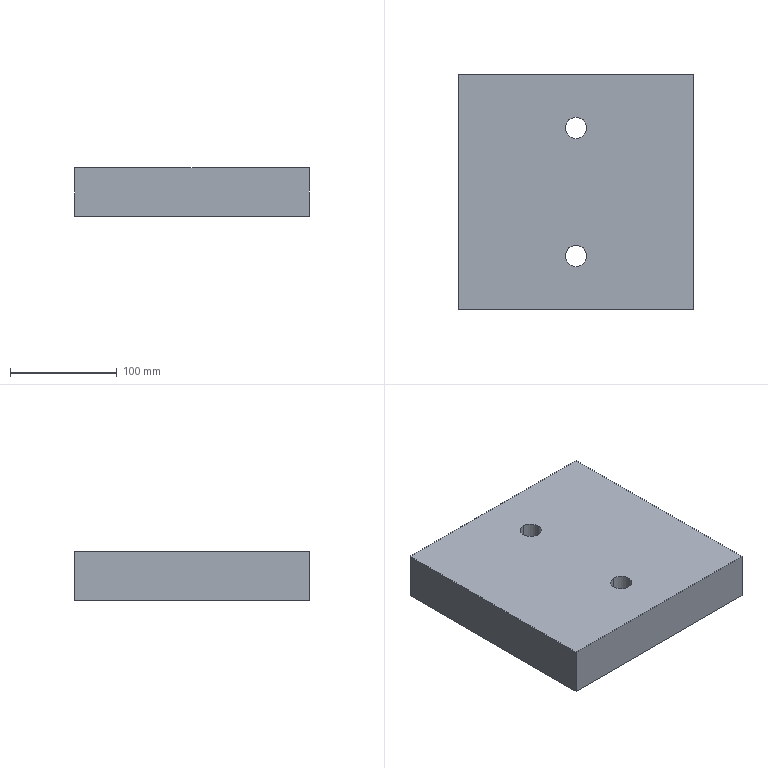Component | SolidWorks | Counterweight-10 | 1 solid | 10 faces | box 220 x 220 x 45 mm | volume 2149726 mm3 | plane 6 | cylinder 4 | commonest cylinder face diameters 20 x4
build123d program:
from build123d import *

# Parameters (mm, degrees)
SKETCH1_W           = 220
SKETCH1_H           = 220
SKETCH1_R           = 10
BOSS_EXTRUDE1_DEPTH = 45


with BuildPart() as part:
    # Sketch1 → Boss-Extrude1 (new body)
    with BuildSketch(Plane.XY):
        Rectangle(SKETCH1_W, SKETCH1_H)
        with Locations(Location((-60, 0, 0), (0, 0, 180))):
            Circle(SKETCH1_R, mode=Mode.SUBTRACT)
        with Locations(Location((60, 0, 0), (0, 0, 180))):
            Circle(SKETCH1_R, mode=Mode.SUBTRACT)
    extrude(amount=BOSS_EXTRUDE1_DEPTH)


solid = part.part

# Placed as in the assembly
solid = solid.moved(Location((-917, -288, -420), (0, 0, 90)))
STEP:
#1=COLOUR_RGB('',0.7922,0.8196,0.9333);
#2=FILL_AREA_STYLE_COLOUR('',#1);
#3=FILL_AREA_STYLE('',(#2));
#4=SURFACE_STYLE_FILL_AREA(#3);
#5=SURFACE_SIDE_STYLE('',(#4));
#6=SURFACE_STYLE_USAGE(.BOTH.,#5);
#7=PRESENTATION_STYLE_ASSIGNMENT((#6));
#8=CARTESIAN_POINT('',(-36.102,-13.307,-16.535));
#9=VERTEX_POINT('',#8);
#10=CARTESIAN_POINT('',(-36.102,-14.094,-16.535));
#11=VERTEX_POINT('',#10);
#12=CARTESIAN_POINT('',(-36.102,-13.701,-16.535));
#13=DIRECTION('',(-0.,-0.,-1.));
#14=DIRECTION('',(0.,1.,0.));
#15=AXIS2_PLACEMENT_3D('',#12,#13,#14);
#16=CIRCLE('',#15,0.3937);
#17=EDGE_CURVE('',#9,#11,#16,.T.);
#18=ORIENTED_EDGE('',*,*,#17,.T.);
#19=CARTESIAN_POINT('',(-36.102,-14.094,-14.764));
#20=VERTEX_POINT('',#19);
#21=CARTESIAN_POINT('',(-36.102,-14.094,-16.535));
#22=DIRECTION('',(0.,0.,1.));
#23=VECTOR('',#22,39.37);
#24=LINE('',#21,#23);
#25=EDGE_CURVE('',#11,#20,#24,.T.);
#26=ORIENTED_EDGE('',*,*,#25,.T.);
#27=CARTESIAN_POINT('',(-36.102,-13.307,-14.764));
#28=VERTEX_POINT('',#27);
#29=CARTESIAN_POINT('',(-36.102,-13.701,-14.764));
#30=DIRECTION('',(-0.,-0.,-1.));
#31=DIRECTION('',(0.,1.,0.));
#32=AXIS2_PLACEMENT_3D('',#29,#30,#31);
#33=CIRCLE('',#32,0.3937);
#34=EDGE_CURVE('',#28,#20,#33,.T.);
#35=ORIENTED_EDGE('',*,*,#34,.F.);
#36=CARTESIAN_POINT('',(-36.102,-13.307,-16.535));
#37=DIRECTION('',(0.,0.,1.));
#38=VECTOR('',#37,39.37);
#39=LINE('',#36,#38);
#40=EDGE_CURVE('',#9,#28,#39,.T.);
#41=ORIENTED_EDGE('',*,*,#40,.F.);
#42=EDGE_LOOP('',(#18,#26,#35,#41));
#43=FACE_OUTER_BOUND('',#42,.T.);
#44=CARTESIAN_POINT('',(-36.102,-13.701,-16.535));
#45=DIRECTION('',(0.,0.,1.));
#46=DIRECTION('',(0.,1.,0.));
#47=AXIS2_PLACEMENT_3D('',#44,#45,#46);
#48=CYLINDRICAL_SURFACE('',#47,0.3937);
#49=ADVANCED_FACE('',(#43),#48,.F.);
#50=CARTESIAN_POINT('',(-36.102,-8.583,-16.535));
#51=VERTEX_POINT('',#50);
#52=CARTESIAN_POINT('',(-36.102,-9.37,-16.535));
#53=VERTEX_POINT('',#52);
#54=CARTESIAN_POINT('',(-36.102,-8.976,-16.535));
#55=DIRECTION('',(-0.,-0.,-1.));
#56=DIRECTION('',(0.,-1.,0.));
#57=AXIS2_PLACEMENT_3D('',#54,#55,#56);
#58=CIRCLE('',#57,0.3937);
#59=EDGE_CURVE('',#51,#53,#58,.T.);
#60=ORIENTED_EDGE('',*,*,#59,.T.);
#61=CARTESIAN_POINT('',(-36.102,-9.37,-14.764));
#62=VERTEX_POINT('',#61);
#63=CARTESIAN_POINT('',(-36.102,-9.37,-16.535));
#64=DIRECTION('',(0.,0.,1.));
#65=VECTOR('',#64,39.37);
#66=LINE('',#63,#65);
#67=EDGE_CURVE('',#53,#62,#66,.T.);
#68=ORIENTED_EDGE('',*,*,#67,.T.);
#69=CARTESIAN_POINT('',(-36.102,-8.583,-14.764));
#70=VERTEX_POINT('',#69);
#71=CARTESIAN_POINT('',(-36.102,-8.976,-14.764));
#72=DIRECTION('',(-0.,-0.,-1.));
#73=DIRECTION('',(0.,-1.,0.));
#74=AXIS2_PLACEMENT_3D('',#71,#72,#73);
#75=CIRCLE('',#74,0.3937);
#76=EDGE_CURVE('',#70,#62,#75,.T.);
#77=ORIENTED_EDGE('',*,*,#76,.F.);
#78=CARTESIAN_POINT('',(-36.102,-8.583,-16.535));
#79=DIRECTION('',(0.,0.,1.));
#80=VECTOR('',#79,39.37);
#81=LINE('',#78,#80);
#82=EDGE_CURVE('',#51,#70,#81,.T.);
#83=ORIENTED_EDGE('',*,*,#82,.F.);
#84=EDGE_LOOP('',(#60,#68,#77,#83));
#85=FACE_OUTER_BOUND('',#84,.T.);
#86=CARTESIAN_POINT('',(-36.102,-8.976,-16.535));
#87=DIRECTION('',(0.,0.,1.));
#88=DIRECTION('',(0.,1.,0.));
#89=AXIS2_PLACEMENT_3D('',#86,#87,#88);
#90=CYLINDRICAL_SURFACE('',#89,0.3937);
#91=ADVANCED_FACE('',(#85),#90,.F.);
#92=ORIENTED_EDGE('',*,*,#59,.F.);
#93=CARTESIAN_POINT('',(-36.102,-8.976,-16.535));
#94=DIRECTION('',(-0.,-0.,-1.));
#95=DIRECTION('',(0.,-1.,0.));
#96=AXIS2_PLACEMENT_3D('',#93,#94,#95);
#97=CIRCLE('',#96,0.3937);
#98=EDGE_CURVE('',#53,#51,#97,.T.);
#99=ORIENTED_EDGE('',*,*,#98,.F.);
#100=EDGE_LOOP('',(#92,#99));
#101=FACE_BOUND('',#100,.T.);
#102=CARTESIAN_POINT('',(-31.772,-15.669,-16.535));
#103=VERTEX_POINT('',#102);
#104=CARTESIAN_POINT('',(-40.433,-15.669,-16.535));
#105=VERTEX_POINT('',#104);
#106=CARTESIAN_POINT('',(-31.772,-15.669,-16.535));
#107=DIRECTION('',(-1.,0.,0.));
#108=VECTOR('',#107,39.37);
#109=LINE('',#106,#108);
#110=EDGE_CURVE('',#103,#105,#109,.T.);
#111=ORIENTED_EDGE('',*,*,#110,.T.);
#112=CARTESIAN_POINT('',(-40.433,-7.008,-16.535));
#113=VERTEX_POINT('',#112);
#114=CARTESIAN_POINT('',(-40.433,-7.008,-16.535));
#115=DIRECTION('',(0.,1.,-0.));
#116=VECTOR('',#115,39.37);
#117=LINE('',#114,#116);
#118=EDGE_CURVE('',#105,#113,#117,.T.);
#119=ORIENTED_EDGE('',*,*,#118,.T.);
#120=CARTESIAN_POINT('',(-31.772,-7.008,-16.535));
#121=VERTEX_POINT('',#120);
#122=CARTESIAN_POINT('',(-31.772,-7.008,-16.535));
#123=DIRECTION('',(1.,-0.,-0.));
#124=VECTOR('',#123,39.37);
#125=LINE('',#122,#124);
#126=EDGE_CURVE('',#113,#121,#125,.T.);
#127=ORIENTED_EDGE('',*,*,#126,.T.);
#128=CARTESIAN_POINT('',(-31.772,-7.008,-16.535));
#129=DIRECTION('',(-0.,-1.,0.));
#130=VECTOR('',#129,39.37);
#131=LINE('',#128,#130);
#132=EDGE_CURVE('',#121,#103,#131,.T.);
#133=ORIENTED_EDGE('',*,*,#132,.T.);
#134=EDGE_LOOP('',(#111,#119,#127,#133));
#135=FACE_OUTER_BOUND('',#134,.T.);
#136=ORIENTED_EDGE('',*,*,#17,.F.);
#137=CARTESIAN_POINT('',(-36.102,-13.701,-16.535));
#138=DIRECTION('',(-0.,-0.,-1.));
#139=DIRECTION('',(0.,1.,0.));
#140=AXIS2_PLACEMENT_3D('',#137,#138,#139);
#141=CIRCLE('',#140,0.3937);
#142=EDGE_CURVE('',#11,#9,#141,.T.);
#143=ORIENTED_EDGE('',*,*,#142,.F.);
#144=EDGE_LOOP('',(#136,#143));
#145=FACE_BOUND('',#144,.T.);
#146=CARTESIAN_POINT('',(-36.102,-11.339,-16.535));
#147=DIRECTION('',(0.,0.,1.));
#148=DIRECTION('',(0.,1.,-0.));
#149=AXIS2_PLACEMENT_3D('',#146,#147,#148);
#150=PLANE('',#149);
#151=ADVANCED_FACE('',(#101,#135,#145),#150,.F.);
#152=ORIENTED_EDGE('',*,*,#76,.T.);
#153=CARTESIAN_POINT('',(-36.102,-8.976,-14.764));
#154=DIRECTION('',(-0.,-0.,-1.));
#155=DIRECTION('',(0.,-1.,0.));
#156=AXIS2_PLACEMENT_3D('',#153,#154,#155);
#157=CIRCLE('',#156,0.3937);
#158=EDGE_CURVE('',#62,#70,#157,.T.);
#159=ORIENTED_EDGE('',*,*,#158,.T.);
#160=EDGE_LOOP('',(#152,#159));
#161=FACE_BOUND('',#160,.T.);
#162=CARTESIAN_POINT('',(-31.772,-15.669,-14.764));
#163=VERTEX_POINT('',#162);
#164=CARTESIAN_POINT('',(-40.433,-15.669,-14.764));
#165=VERTEX_POINT('',#164);
#166=CARTESIAN_POINT('',(-31.772,-15.669,-14.764));
#167=DIRECTION('',(-1.,0.,0.));
#168=VECTOR('',#167,39.37);
#169=LINE('',#166,#168);
#170=EDGE_CURVE('',#163,#165,#169,.T.);
#171=ORIENTED_EDGE('',*,*,#170,.F.);
#172=CARTESIAN_POINT('',(-31.772,-7.008,-14.764));
#173=VERTEX_POINT('',#172);
#174=CARTESIAN_POINT('',(-31.772,-7.008,-14.764));
#175=DIRECTION('',(-0.,-1.,0.));
#176=VECTOR('',#175,39.37);
#177=LINE('',#174,#176);
#178=EDGE_CURVE('',#173,#163,#177,.T.);
#179=ORIENTED_EDGE('',*,*,#178,.F.);
#180=CARTESIAN_POINT('',(-40.433,-7.008,-14.764));
#181=VERTEX_POINT('',#180);
#182=CARTESIAN_POINT('',(-31.772,-7.008,-14.764));
#183=DIRECTION('',(1.,-0.,-0.));
#184=VECTOR('',#183,39.37);
#185=LINE('',#182,#184);
#186=EDGE_CURVE('',#181,#173,#185,.T.);
#187=ORIENTED_EDGE('',*,*,#186,.F.);
#188=CARTESIAN_POINT('',(-40.433,-7.008,-14.764));
#189=DIRECTION('',(0.,1.,-0.));
#190=VECTOR('',#189,39.37);
#191=LINE('',#188,#190);
#192=EDGE_CURVE('',#165,#181,#191,.T.);
#193=ORIENTED_EDGE('',*,*,#192,.F.);
#194=EDGE_LOOP('',(#171,#179,#187,#193));
#195=FACE_OUTER_BOUND('',#194,.T.);
#196=ORIENTED_EDGE('',*,*,#34,.T.);
#197=CARTESIAN_POINT('',(-36.102,-13.701,-14.764));
#198=DIRECTION('',(-0.,-0.,-1.));
#199=DIRECTION('',(0.,1.,0.));
#200=AXIS2_PLACEMENT_3D('',#197,#198,#199);
#201=CIRCLE('',#200,0.3937);
#202=EDGE_CURVE('',#20,#28,#201,.T.);
#203=ORIENTED_EDGE('',*,*,#202,.T.);
#204=EDGE_LOOP('',(#196,#203));
#205=FACE_BOUND('',#204,.T.);
#206=CARTESIAN_POINT('',(-36.102,-11.339,-14.764));
#207=DIRECTION('',(0.,0.,1.));
#208=DIRECTION('',(0.,1.,-0.));
#209=AXIS2_PLACEMENT_3D('',#206,#207,#208);
#210=PLANE('',#209);
#211=ADVANCED_FACE('',(#161,#195,#205),#210,.T.);
#212=ORIENTED_EDGE('',*,*,#170,.T.);
#213=CARTESIAN_POINT('',(-40.433,-15.669,-16.535));
#214=DIRECTION('',(0.,0.,1.));
#215=VECTOR('',#214,39.37);
#216=LINE('',#213,#215);
#217=EDGE_CURVE('',#105,#165,#216,.T.);
#218=ORIENTED_EDGE('',*,*,#217,.F.);
#219=ORIENTED_EDGE('',*,*,#110,.F.);
#220=CARTESIAN_POINT('',(-31.772,-15.669,-16.535));
#221=DIRECTION('',(0.,0.,1.));
#222=VECTOR('',#221,39.37);
#223=LINE('',#220,#222);
#224=EDGE_CURVE('',#103,#163,#223,.T.);
#225=ORIENTED_EDGE('',*,*,#224,.T.);
#226=EDGE_LOOP('',(#212,#218,#219,#225));
#227=FACE_OUTER_BOUND('',#226,.T.);
#228=CARTESIAN_POINT('',(-31.772,-15.669,-16.535));
#229=DIRECTION('',(0.,1.,-0.));
#230=DIRECTION('',(-0.,-0.,-1.));
#231=AXIS2_PLACEMENT_3D('',#228,#229,#230);
#232=PLANE('',#231);
#233=ADVANCED_FACE('',(#227),#232,.F.);
#234=ORIENTED_EDGE('',*,*,#192,.T.);
#235=CARTESIAN_POINT('',(-40.433,-7.008,-16.535));
#236=DIRECTION('',(0.,0.,1.));
#237=VECTOR('',#236,39.37);
#238=LINE('',#235,#237);
#239=EDGE_CURVE('',#113,#181,#238,.T.);
#240=ORIENTED_EDGE('',*,*,#239,.F.);
#241=ORIENTED_EDGE('',*,*,#118,.F.);
#242=ORIENTED_EDGE('',*,*,#217,.T.);
#243=EDGE_LOOP('',(#234,#240,#241,#242));
#244=FACE_OUTER_BOUND('',#243,.T.);
#245=CARTESIAN_POINT('',(-40.433,-7.008,-16.535));
#246=DIRECTION('',(1.,-0.,-0.));
#247=DIRECTION('',(0.,0.,1.));
#248=AXIS2_PLACEMENT_3D('',#245,#246,#247);
#249=PLANE('',#248);
#250=ADVANCED_FACE('',(#244),#249,.F.);
#251=ORIENTED_EDGE('',*,*,#186,.T.);
#252=CARTESIAN_POINT('',(-31.772,-7.008,-16.535));
#253=DIRECTION('',(0.,0.,1.));
#254=VECTOR('',#253,39.37);
#255=LINE('',#252,#254);
#256=EDGE_CURVE('',#121,#173,#255,.T.);
#257=ORIENTED_EDGE('',*,*,#256,.F.);
#258=ORIENTED_EDGE('',*,*,#126,.F.);
#259=ORIENTED_EDGE('',*,*,#239,.T.);
#260=EDGE_LOOP('',(#251,#257,#258,#259));
#261=FACE_OUTER_BOUND('',#260,.T.);
#262=CARTESIAN_POINT('',(-31.772,-7.008,-16.535));
#263=DIRECTION('',(-0.,-1.,0.));
#264=DIRECTION('',(0.,0.,1.));
#265=AXIS2_PLACEMENT_3D('',#262,#263,#264);
#266=PLANE('',#265);
#267=ADVANCED_FACE('',(#261),#266,.F.);
#268=ORIENTED_EDGE('',*,*,#178,.T.);
#269=ORIENTED_EDGE('',*,*,#224,.F.);
#270=ORIENTED_EDGE('',*,*,#132,.F.);
#271=ORIENTED_EDGE('',*,*,#256,.T.);
#272=EDGE_LOOP('',(#268,#269,#270,#271));
#273=FACE_OUTER_BOUND('',#272,.T.);
#274=CARTESIAN_POINT('',(-31.772,-7.008,-16.535));
#275=DIRECTION('',(-1.,0.,0.));
#276=DIRECTION('',(-0.,-0.,-1.));
#277=AXIS2_PLACEMENT_3D('',#274,#275,#276);
#278=PLANE('',#277);
#279=ADVANCED_FACE('',(#273),#278,.F.);
#280=ORIENTED_EDGE('',*,*,#67,.F.);
#281=ORIENTED_EDGE('',*,*,#98,.T.);
#282=ORIENTED_EDGE('',*,*,#82,.T.);
#283=ORIENTED_EDGE('',*,*,#158,.F.);
#284=EDGE_LOOP('',(#280,#281,#282,#283));
#285=FACE_OUTER_BOUND('',#284,.T.);
#286=CARTESIAN_POINT('',(-36.102,-8.976,-16.535));
#287=DIRECTION('',(0.,0.,1.));
#288=DIRECTION('',(0.,1.,0.));
#289=AXIS2_PLACEMENT_3D('',#286,#287,#288);
#290=CYLINDRICAL_SURFACE('',#289,0.3937);
#291=ADVANCED_FACE('',(#285),#290,.F.);
#292=ORIENTED_EDGE('',*,*,#25,.F.);
#293=ORIENTED_EDGE('',*,*,#142,.T.);
#294=ORIENTED_EDGE('',*,*,#40,.T.);
#295=ORIENTED_EDGE('',*,*,#202,.F.);
#296=EDGE_LOOP('',(#292,#293,#294,#295));
#297=FACE_OUTER_BOUND('',#296,.T.);
#298=CARTESIAN_POINT('',(-36.102,-13.701,-16.535));
#299=DIRECTION('',(0.,0.,1.));
#300=DIRECTION('',(0.,1.,0.));
#301=AXIS2_PLACEMENT_3D('',#298,#299,#300);
#302=CYLINDRICAL_SURFACE('',#301,0.3937);
#303=ADVANCED_FACE('',(#297),#302,.F.);
#304=CLOSED_SHELL('',(#49,#91,#151,#211,#233,#250,#267,#279,#291,#303));
#305=MANIFOLD_SOLID_BREP('',#304);
#306=STYLED_ITEM('',(#7),#305);
#307=(LENGTH_UNIT()NAMED_UNIT(*)SI_UNIT($,.METRE.));
#308=LENGTH_MEASURE_WITH_UNIT(LENGTH_MEASURE(0.0254),#307);
#309=DIMENSIONAL_EXPONENTS(1.,0.,0.,0.,0.,0.,0.);
#310=(CONVERSION_BASED_UNIT('',#308)LENGTH_UNIT()NAMED_UNIT(#309));
#311=UNCERTAINTY_MEASURE_WITH_UNIT(LENGTH_MEASURE(0.00001),#310,'','');
#312=(NAMED_UNIT(*)PLANE_ANGLE_UNIT()SI_UNIT($,.RADIAN.));
#313=(NAMED_UNIT(*)SI_UNIT($,.STERADIAN.)SOLID_ANGLE_UNIT());
#314=(GEOMETRIC_REPRESENTATION_CONTEXT(3)GLOBAL_UNCERTAINTY_ASSIGNED_CONTEXT((#311))GLOBAL_UNIT_ASSIGNED_CONTEXT((#310,#312,#313))REPRESENTATION_CONTEXT('',''));
#315=MECHANICAL_DESIGN_GEOMETRIC_PRESENTATION_REPRESENTATION('',(#306),#314);
#316=CARTESIAN_POINT('',(0.,0.,0.));
#317=DIRECTION('',(0.,0.,1.));
#318=DIRECTION('',(1.,0.,0.));
#319=AXIS2_PLACEMENT_3D('',#316,#317,#318);
#320=(LENGTH_UNIT()NAMED_UNIT(*)SI_UNIT($,.METRE.));
#321=LENGTH_MEASURE_WITH_UNIT(LENGTH_MEASURE(0.0254),#320);
#322=DIMENSIONAL_EXPONENTS(1.,0.,0.,0.,0.,0.,0.);
#323=(CONVERSION_BASED_UNIT('',#321)LENGTH_UNIT()NAMED_UNIT(#322));
#324=UNCERTAINTY_MEASURE_WITH_UNIT(LENGTH_MEASURE(0.00001),#323,'','');
#325=(NAMED_UNIT(*)PLANE_ANGLE_UNIT()SI_UNIT($,.RADIAN.));
#326=(NAMED_UNIT(*)SI_UNIT($,.STERADIAN.)SOLID_ANGLE_UNIT());
#327=(GEOMETRIC_REPRESENTATION_CONTEXT(3)GLOBAL_UNCERTAINTY_ASSIGNED_CONTEXT((#324))GLOBAL_UNIT_ASSIGNED_CONTEXT((#323,#325,#326))REPRESENTATION_CONTEXT('',''));
#328=ADVANCED_BREP_SHAPE_REPRESENTATION('',(#305,#319),#327);
#329=PRESENTATION_LAYER_ASSIGNMENT('','',(#306));